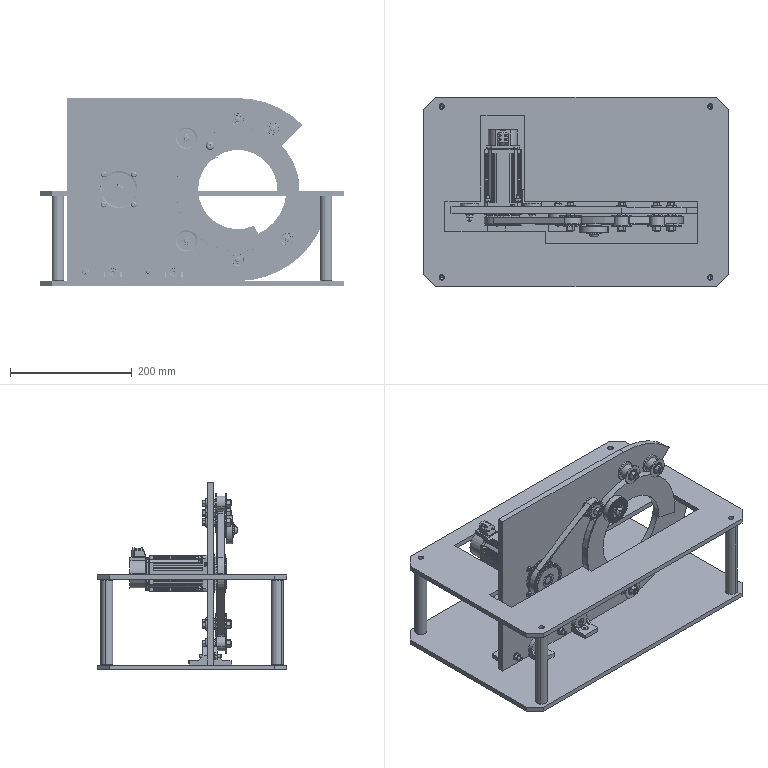Assembly | SolidWorks | mm | 79 component files | 79 solids | 3945 faces | box 500 x 310 x 308 mm | volume 3994242 mm3 | plane 1205 | cylinder 1120 | sphere 580 | torus 521 | cone 493 | spline 26 | commonest cylinder face diameters 0.4 x216 3.86 x111 17.1 x64 8 x48 30.69 x40 9 x36 56.16 x36 19 x32
Bill of materials:
60-90SeriesServoMotor[60ST-M00630]_60ST-M00630 | 1 |  | Elongated prismatic body with a square front flange, a protruding stepped cylindrical shaft, a cylindrical rear section, and a raised block on top of the rear section. Overall the shape looks like an electric motor.
AdhesiveTape | 1 |  | Flat strip wound into a tight planar spiral of many turns, with an open central hole and a free outer end. It looks like a coiled strip or a spiral spring.
AdhesiveTapeRoll | 1 |  | Spool or bobbin shape: a cylindrical tube with a thin disc flange at each end and a through bore.
ArcToothIdlerBearingTypeAtBothEnds[ST5GTD-20-12-Q]_ST5GTD-20-12-Q | 2 |  | Toothed pulley with a flange at each end, a relatively small number of coarse axial teeth, a short hub boss on each face, and a plain round through bore.
ArcToothIdlerBearingTypeAtBothEnds[ST5GTD-36-15-Q]_ST5GTD-36-15-Q | 1 |  | Toothed pulley with a flange at each end, many fine axial teeth, a shallow hub boss on the faces, and a through bore with a single keyway.
Belt2 | 1 |  | Thin closed band forming a rounded triangular loop with one concave side. It looks like a belt shown wrapped along a path around several rounded points.
Column | 4 |  | Long slender cylindrical tube or rod with a small coaxial bore at the end. The tessellated end view shows a faceted conical surface inside the bore.
FixedPlate | 1 |  | Flat plate, mostly rectangular with one rounded end. A large circular cutout opens to the edge through an angled slot, giving a C-shaped opening. The plate has several small through-holes.
FixedPlateA | 1 |  | Flat rectangular plate with chamfered corners, four corner holes, and a large irregular stepped through-cutout shaped roughly like an inverted T or L.
FixedPlateB | 1 |  | Flat rectangular plate with chamfered corners, four corner holes, and four smaller holes in a skewed quadrilateral group toward one side.
FlatWasher_6 | 4 | Plain Carbon Steel | Flat annular ring, washer-like, with a plain round center hole and flat parallel faces.
FlatWasher_8 | 1 | Plain Carbon Steel | Thin flat annular ring, washer-like, with a plain round center hole and flat parallel faces.
GB_T16674-1996HexagonHeadFlangeBolt(SmallSeries)M8_40 | 6 |  | Headed shaft with a hexagonal head and an integral round flange (rounded edge) under the head, a long plain cylindrical shank, and a chamfered tip; looks like a hex flange bolt.
GB_T41-2000Type1HexNutGradeCM8 | 6 |  | Tall hexagonal nut-like body with a plain through bore. Its axial length is greater than its across-flats width. The corners are chamfered, so arcs show on the flats.
GB_T6172.1-2000HexThinNutGradeAAndBM8 | 6 |  | Thin hexagonal nut-like body with a large through bore that has a chamfered or countersunk entry. The corners are chamfered on the end faces.
HexNutM5 | 4 |  | Hexagonal nut-like body with a plain through bore. Both ends are chamfered, giving curved arcs on each flat.
HexNutM6 | 4 |  | Hexagonal nut-like body with a plain through bore. Both ends are chamfered, with curved arcs on the flats.
BearingSleeve | 4 |  | Spool-shaped, axisymmetric body: a cylindrical hub between two thin end flanges with chamfered edges. It has a central through bore with a stepped or counterbored entry at the end.
GB_T276-94DeepGrooveBallBearing62800-2Z | 8 |  | Annular body with an outer ring and an inner ring. Rolling elements that look like balls are visible in the gap between the rings. It looks like a ball bearing without shields.
SocketCountersunkHeadScrewM6x30 | 4 |  | Long plain cylindrical shank with a conical countersunk head at one end and a chamfered tip at the other.
SocketCountersunkHeadScrewM6x8 | 4 |  | Short countersunk-head fastener-like part with a hexagonal socket recess in the flat head top, a short cylindrical shank, and a chamfered end.
SocketHeadCapScrewM5x30 | 4 | Plain Carbon Steel | Long fastener-like part with a domed (button) head that has a hexagonal socket recess, a long plain cylindrical shank, and a chamfered tip.
SocketHeadCapScrewM8x20 | 1 | Plain Carbon Steel | Short fastener-like part with a domed (button) head that has a hexagonal socket recess, a plain cylindrical shank, and a chamfered tip.
SpringWasher_5 | 4 | Plain Carbon Steel | Split ring with a rectangular cross-section and one radial gap. It looks like a split lock washer.
TurningAnglePieceHDH[HDH-83030]_HDH-83030 | 4 |  | L-shaped angle bracket. A rectangular base plate meets an upright plate with a semicircular top. Each plate has one countersunk through-hole, and a triangular gusset sits on each side where the plates meet.
Turntable | 1 |  | Thin, flat, open split ring (C-shape) with a uniform rectangular cross-section. It has one angled gap cut through the ring and one small round hole near the outer edge.
Mates:
1. concentric | 60-90SeriesServoMotor[60ST-M00630]_60ST-M00630-1 face at (-120, -55, 158) dir (0, -1, 0) r 7 | ArcToothIdlerBearingTypeAtBothEnds[ST5GTD-36-15-Q]_ST5GTD-36-15-Q-1 face at (-120, 4.15, 158) dir (0, -1, 0) r 7.5
2. coincident | 60-90SeriesServoMotor[60ST-M00630]_60ST-M00630-1 face at (-120, -55, 165) dir (0, -1, 0) | ArcToothIdlerBearingTypeAtBothEnds[ST5GTD-36-15-Q]_ST5GTD-36-15-Q-1 face at (-115.053, -55, 134.005) dir (0, -1, 0)
3. concentric | ArcToothIdlerBearingTypeAtBothEnds[ST5GTD-20-12-Q]_ST5GTD-20-12-Q-1 face at (-9.146, -42.5, 242.146) dir (0, -1, 0) r 5.5 | GB_T16674-1996HexagonHeadFlangeBolt(SmallSeries)M8_40-3 face at (-9.146, -65, 242.146) dir (0, 1, 0) r 4
4. coincident | ArcToothIdlerBearingTypeAtBothEnds[ST5GTD-20-12-Q]_ST5GTD-20-12-Q-1 face at (-7.098, -56, 237.041) dir (0, -1, 0) | GB_T41-2000Type1HexNutGradeCM8-3 face at (1.931, -56, 236.804) dir (0, 1, 0)
5. concentric | ArcToothIdlerBearingTypeAtBothEnds[ST5GTD-20-12-Q]_ST5GTD-20-12-Q-2 face at (-9.146, 2.5, 73.854) dir (0, -1, 0) r 4 | GB_T16674-1996HexagonHeadFlangeBolt(SmallSeries)M8_40-4 face at (-9.146, -65, 73.854) dir (0, 1, 0) r 4
6. coincident | ArcToothIdlerBearingTypeAtBothEnds[ST5GTD-20-12-Q]_ST5GTD-20-12-Q-2 face at (-11.865, -56, 69.073) dir (0, -1, 0) | GB_T41-2000Type1HexNutGradeCM8-4 face at (1.931, -56, 68.513) dir (0, 1, 0)
7. concentric | FixedPlate-1 face at (75, -25, 158) dir (0, -1, 0) r 80 | Turntable-1 face at (75, -40.5, 158) dir (0, -1, 0) r 65
8. coincident | Roller-1/BearingSleeve-1 face at (75, -40.5, 273) dir (0, -1, 0) | Turntable-1 face at (75, -40.5, 158) dir (0, 1, 0)
9. coincident | FixedPlate-1 face at (0, -35, 158) dir (0, -1, 0) | SocketHeadCapScrewM5x30-1 plane at (-95.251, -35, 133.251) dir (0, 1, 0)
10. coincident | 60-90SeriesServoMotor[60ST-M00630]_60ST-M00630-1 face at (-144.5, -17, 133.5) dir (0, 1, 0) | SpringWasher_5-1 plane at (-95.251, -17, 133.251) dir (0, -1, 0)
11. coincident | HexNutM5-1 plane at (-95.251, -15.8, 133.251) dir (0, -1, 0) | SpringWasher_5-1 plane at (-95.251, -15.8, 133.251) dir (0, 1, 0)
12. concentric | 60-90SeriesServoMotor[60ST-M00630]_60ST-M00630-1 face at (-95.251, 70.251, 133.251) dir (0, -1, 0) r 2.75 | SocketHeadCapScrewM5x30-1 axis at (-95.251, -37.5, 133.251) dir (0, 1, 0)
13. coincident | HexNutM5-1 axis at (-95.251, -15.8, 133.251) dir (0, 1, 0) | SocketHeadCapScrewM5x30-1 axis at (-95.251, -37.5, 133.251) dir (0, 1, 0)
14. coincident | SpringWasher_5-1 axis at (-95.251, -15.8, 133.251) dir (0, -1, 0) | SocketHeadCapScrewM5x30-1 axis at (-95.251, -37.5, 133.251) dir (0, 1, 0)
15. coincident | SpringWasher_5-2 plane at (-144.749, -15.8, 133.251) dir (0, 1, 0) | HexNutM5-2 plane at (-144.749, -15.8, 133.251) dir (0, -1, 0)
16. coincident | SocketHeadCapScrewM5x30-2 axis at (-144.749, -37.5, 133.251) dir (0, 1, 0) | HexNutM5-2 axis at (-144.749, -15.8, 133.251) dir (0, 1, 0)
17. coincident | SocketHeadCapScrewM5x30-2 axis at (-144.749, -37.5, 133.251) dir (0, 1, 0) | SpringWasher_5-2 axis at (-144.749, -15.8, 133.251) dir (0, -1, 0)
18. coincident | FixedPlate-1 face at (0, -35, 158) dir (0, -1, 0) | SocketHeadCapScrewM5x30-2 plane at (-144.749, -35, 133.251) dir (0, 1, 0)
19. coincident | 60-90SeriesServoMotor[60ST-M00630]_60ST-M00630-1 face at (-144.5, -17, 133.5) dir (0, 1, 0) | SpringWasher_5-2 plane at (-144.749, -17, 133.251) dir (0, -1, 0)
20. concentric | 60-90SeriesServoMotor[60ST-M00630]_60ST-M00630-1 face at (-144.749, 70.251, 133.251) dir (0, -1, 0) r 2.75 | SocketHeadCapScrewM5x30-2 axis at (-144.749, -37.5, 133.251) dir (0, 1, 0)
21. coincident | SpringWasher_5-3 plane at (-144.749, -15.8, 182.749) dir (0, 1, 0) | HexNutM5-3 plane at (-144.749, -15.8, 182.749) dir (0, -1, 0)
22. coincident | SocketHeadCapScrewM5x30-3 axis at (-144.749, -37.5, 182.749) dir (0, 1, 0) | HexNutM5-3 axis at (-144.749, -15.8, 182.749) dir (0, 1, 0)
23. coincident | SocketHeadCapScrewM5x30-3 axis at (-144.749, -37.5, 182.749) dir (0, 1, 0) | SpringWasher_5-3 axis at (-144.749, -15.8, 182.749) dir (0, -1, 0)
24. coincident | FixedPlate-1 face at (0, -35, 158) dir (0, -1, 0) | SocketHeadCapScrewM5x30-3 plane at (-144.749, -35, 182.749) dir (0, 1, 0)
25. coincident | 60-90SeriesServoMotor[60ST-M00630]_60ST-M00630-1 face at (-144.5, -17, 133.5) dir (0, 1, 0) | SpringWasher_5-3 plane at (-144.749, -17, 182.749) dir (0, -1, 0)
26. concentric | 60-90SeriesServoMotor[60ST-M00630]_60ST-M00630-1 face at (-144.749, 70.251, 182.749) dir (0, -1, 0) r 2.75 | SocketHeadCapScrewM5x30-3 axis at (-144.749, -37.5, 182.749) dir (0, 1, 0)
27. coincident | SpringWasher_5-4 plane at (-95.251, -15.8, 182.749) dir (0, 1, 0) | HexNutM5-4 plane at (-95.251, -15.8, 182.749) dir (0, -1, 0)
28. coincident | SocketHeadCapScrewM5x30-4 axis at (-95.251, -37.5, 182.749) dir (0, 1, 0) | HexNutM5-4 axis at (-95.251, -15.8, 182.749) dir (0, 1, 0)
29. coincident | SocketHeadCapScrewM5x30-4 axis at (-95.251, -37.5, 182.749) dir (0, 1, 0) | SpringWasher_5-4 axis at (-95.251, -15.8, 182.749) dir (0, -1, 0)
30. coincident | FixedPlate-1 face at (0, -35, 158) dir (0, -1, 0) | SocketHeadCapScrewM5x30-4 plane at (-95.251, -35, 182.749) dir (0, 1, 0)
31. coincident | 60-90SeriesServoMotor[60ST-M00630]_60ST-M00630-1 face at (-144.5, -17, 133.5) dir (0, 1, 0) | SpringWasher_5-4 plane at (-95.251, -17, 182.749) dir (0, -1, 0)
32. concentric | 60-90SeriesServoMotor[60ST-M00630]_60ST-M00630-1 face at (-95.251, 70.251, 182.749) dir (0, -1, 0) r 2.75 | SocketHeadCapScrewM5x30-4 axis at (-95.251, -37.5, 182.749) dir (0, 1, 0)
33. coincident | TurningAnglePieceHDH[HDH-83030]_HDH-83030-3 face at (-159.718, -18, 38) dir (0, 1, 0) | SocketCountersunkHeadScrewM6x30-1 plane at (-174.718, -18, 23) dir (0, -1, 0)
34. coincident | FixedPlate-1 face at (0, -35, 158) dir (0, -1, 0) | FlatWasher_6-2 plane at (-174.718, -35, 23) dir (0, 1, 0)
35. coincident | HexNutM6-2 plane at (-174.718, -36.4, 23) dir (0, 1, 0) | FlatWasher_6-2 plane at (-174.718, -36.4, 23) dir (0, -1, 0)
36. concentric | FixedPlate-1 face at (-174.718, -25, 23) dir (0, -1, 0) r 3.25 | SocketCountersunkHeadScrewM6x30-1 axis at (-174.718, -47.4, 23) dir (0, 1, 0)
37. coincident | HexNutM6-2 axis at (-174.718, -36.4, 23) dir (0, -1, 0) | SocketCountersunkHeadScrewM6x30-1 axis at (-174.718, -47.4, 23) dir (0, 1, 0)
38. coincident | FlatWasher_6-2 axis at (-174.718, -36.4, 23) dir (0, 1, 0) | SocketCountersunkHeadScrewM6x30-1 axis at (-174.718, -47.4, 23) dir (0, 1, 0)
39. coincident | TurningAnglePieceHDH[HDH-83030]_HDH-83030-2 face at (-56.946, -18, 38) dir (0, 1, 0) | SocketCountersunkHeadScrewM6x30-2 plane at (-71.946, -18, 23) dir (0, -1, 0)
40. coincident | FixedPlate-1 face at (0, -35, 158) dir (0, -1, 0) | FlatWasher_6-3 plane at (-71.946, -35, 23) dir (0, 1, 0)
41. coincident | HexNutM6-3 plane at (-71.946, -36.4, 23) dir (0, 1, 0) | FlatWasher_6-3 plane at (-71.946, -36.4, 23) dir (0, -1, 0)
42. concentric | FixedPlate-1 face at (-71.946, -25, 23) dir (0, -1, 0) r 3.25 | SocketCountersunkHeadScrewM6x30-2 axis at (-71.946, -47.4, 23) dir (0, 1, 0)
43. coincident | HexNutM6-3 axis at (-71.946, -36.4, 23) dir (0, -1, 0) | SocketCountersunkHeadScrewM6x30-2 axis at (-71.946, -47.4, 23) dir (0, 1, 0)
44. coincident | FlatWasher_6-3 axis at (-71.946, -36.4, 23) dir (0, 1, 0) | SocketCountersunkHeadScrewM6x30-2 axis at (-71.946, -47.4, 23) dir (0, 1, 0)
45. coincident | TurningAnglePieceHDH[HDH-83030]_HDH-83030-4 face at (-145, -42, 38) dir (0, -1, 0) | SocketCountersunkHeadScrewM6x30-3 plane at (-130, -42, 23) dir (0, 1, 0)
46. concentric | FixedPlate-1 face at (-130, -25, 23) dir (0, -1, 0) r 3.25 | SocketCountersunkHeadScrewM6x30-3 axis at (-130, -12.6, 23) dir (0, -1, 0)
47. coincident | TurningAnglePieceHDH[HDH-83030]_HDH-83030-1 face at (-45, -42, 38) dir (0, -1, 0) | SocketCountersunkHeadScrewM6x30-4 plane at (-30, -42, 23) dir (0, 1, 0)
48. concentric | FixedPlate-1 face at (-30, -25, 23) dir (0, -1, 0) r 3.25 | SocketCountersunkHeadScrewM6x30-4 axis at (-30, -12.6, 23) dir (0, -1, 0)
49. concentric | FlatWasher_6-7 face at (-130, -25, 23) dir (0, 1, 0) r 6 | HexNutM6-7 face at (-130, -18.4, 23) dir (0, -1, 0) r 3
50. coincident | FlatWasher_6-7 face at (-130, -23.6, 23) dir (0, 1, 0) | HexNutM6-7 face at (-130, -23.6, 23) dir (0, -1, 0)
51. coincident | FlatWasher_6-6 face at (-30, -23.6, 23) dir (0, 1, 0) | HexNutM6-6 face at (-30, -23.6, 23) dir (0, -1, 0)
52. concentric | FlatWasher_6-6 face at (-30, -25, 23) dir (0, 1, 0) r 3.2 | HexNutM6-6 face at (-30, -18.4, 23) dir (0, -1, 0) r 3
53. concentric | SocketCountersunkHeadScrewM6x30-4 face at (-30, -12, 23) dir (0, -1, 0) r 3 | HexNutM6-6 face at (-30, -18.4, 23) dir (0, -1, 0) r 3
54. coincident | FixedPlate-1 face at (0, -25, 158) dir (0, 1, 0) | FlatWasher_6-6 face at (-30, -25, 23) dir (0, -1, 0)
55. concentric | SocketCountersunkHeadScrewM6x30-3 face at (-130, -12, 23) dir (0, -1, 0) r 3 | HexNutM6-7 face at (-130, -18.4, 23) dir (0, -1, 0) r 3
56. coincident | FixedPlate-1 face at (0, -25, 158) dir (0, 1, 0) | FlatWasher_6-7 face at (-130, -25, 23) dir (0, -1, 0)
57. coincident | TurningAnglePieceHDH[HDH-83030]_HDH-83030-3 face at (-159.718, -18, 15) dir (0, 0, 1) | SocketCountersunkHeadScrewM6x8-1 plane at (-174.718, -10, 15) dir (0, 0, -1)
58. concentric | TurningAnglePieceHDH[HDH-83030]_HDH-83030-3 face at (-174.718, -10, 15) dir (0, 0, 1) r 3.25 | SocketCountersunkHeadScrewM6x8-1 axis at (-174.718, -10, 7.6) dir (0, 0, 1)
59. concentric | TurningAnglePieceHDH[HDH-83030]_HDH-83030-2 face at (-71.946, -10, 15) dir (0, 0, 1) r 3.25 | SocketCountersunkHeadScrewM6x8-3 edge at (-71.946, -10, 15) dir (0, 0, -1) r 5.65
60. coincident | TurningAnglePieceHDH[HDH-83030]_HDH-83030-2 face at (-56.946, -18, 15) dir (0, 0, 1) | SocketCountersunkHeadScrewM6x8-3 face at (-71.946, -10, 15) dir (0, 0, 1)
61. coincident | TurningAnglePieceHDH[HDH-83030]_HDH-83030-4 face at (-145, -42, 15) dir (0, 0, 1) | SocketCountersunkHeadScrewM6x8-5 face at (-130, -50, 15) dir (0, 0, 1)
62. concentric | TurningAnglePieceHDH[HDH-83030]_HDH-83030-4 face at (-130, -50, 15) dir (0, 0, -1) r 785.397 | SocketCountersunkHeadScrewM6x8-5 face at (-130, -50, 11.28) dir (0, 0, -1) r 785.398
63. coincident | TurningAnglePieceHDH[HDH-83030]_HDH-83030-1 face at (-45, -42, 15) dir (0, 0, 1) | SocketCountersunkHeadScrewM6x8-6 face at (-30, -50, 15) dir (0, 0, 1)
64. concentric | TurningAnglePieceHDH[HDH-83030]_HDH-83030-1 face at (-30, -50, 15) dir (0, 0, -1) r 785.397 | SocketCountersunkHeadScrewM6x8-6 face at (-30, -50, 11.28) dir (0, 0, -1) r 785.398
65. concentric | Turntable-1 face at (29.475, -52.5, 229.781) dir (0, -1, 0) r 3.4 | AdhesiveTapeRoll-1 face at (29.475, -68.5, 229.781) dir (0, 1, 0) r 4.2
66. coincident | Turntable-1 face at (75, -52.5, 158) dir (0, -1, 0) | AdhesiveTapeRoll-1 face at (29.475, -52.5, 229.781) dir (0, 1, 0)
67. coincident | AdhesiveTapeRoll-1 face at (34.468, -66.5, 229.511) dir (0, 1, 0) | AdhesiveTape-1 face at (43.009, -66.5, 233.364) dir (0, -1, 0)
68. concentric | AdhesiveTapeRoll-1 face at (29.475, -68.5, 229.781) dir (0, 1, 0) r 4.2 | AdhesiveTape-1 sketch segment at (29.475, -66.5, 229.781) dir (0, 1, 0) r 5
69. coincident | AdhesiveTapeRoll-1 face at (41.457, -68.5, 229.133) dir (0, -1, 0) | FlatWasher_8-1 plane at (29.475, -68.5, 229.781) dir (0, 1, 0)
70. coincident | FlatWasher_8-1 plane at (29.475, -69.9, 229.781) dir (0, -1, 0) | SocketHeadCapScrewM8x20-1 plane at (29.475, -69.9, 229.781) dir (0, 1, 0)
71. concentric | Turntable-1 face at (29.475, -52.5, 229.781) dir (0, -1, 0) r 3.4 | SocketHeadCapScrewM8x20-1 axis at (29.475, -74, 229.781) dir (0, 1, 0)
72. coincident | FlatWasher_8-1 axis at (29.475, -69.9, 229.781) dir (0, 1, 0) | SocketHeadCapScrewM8x20-1 axis at (29.475, -74, 229.781) dir (0, 1, 0)